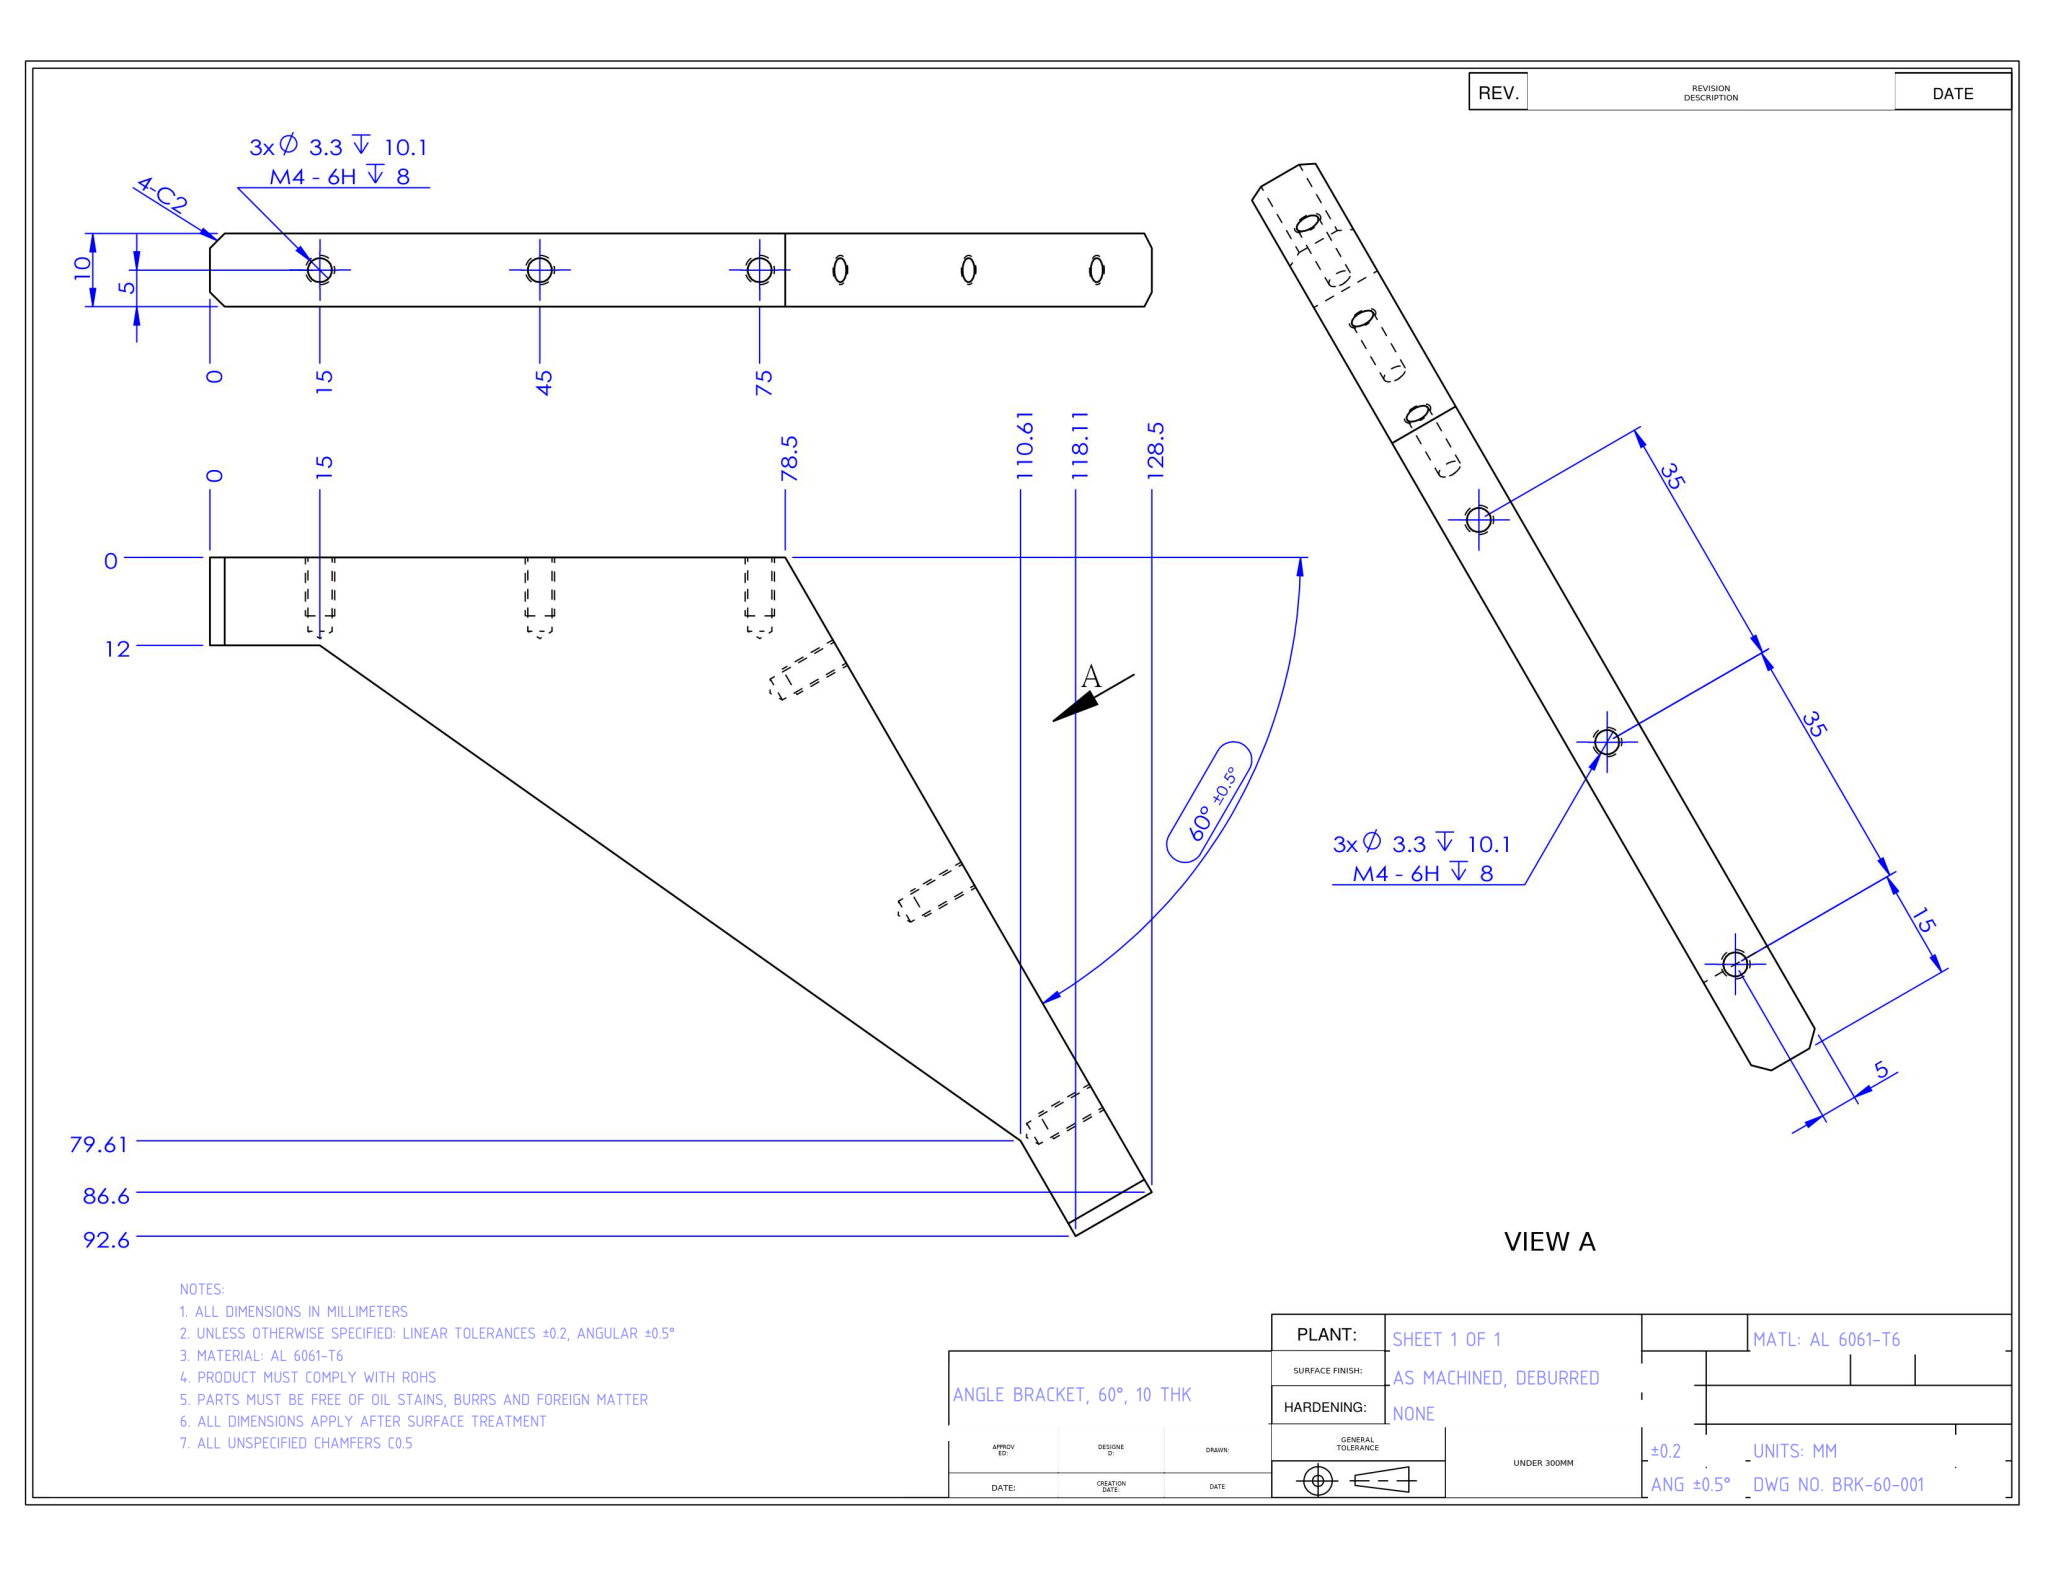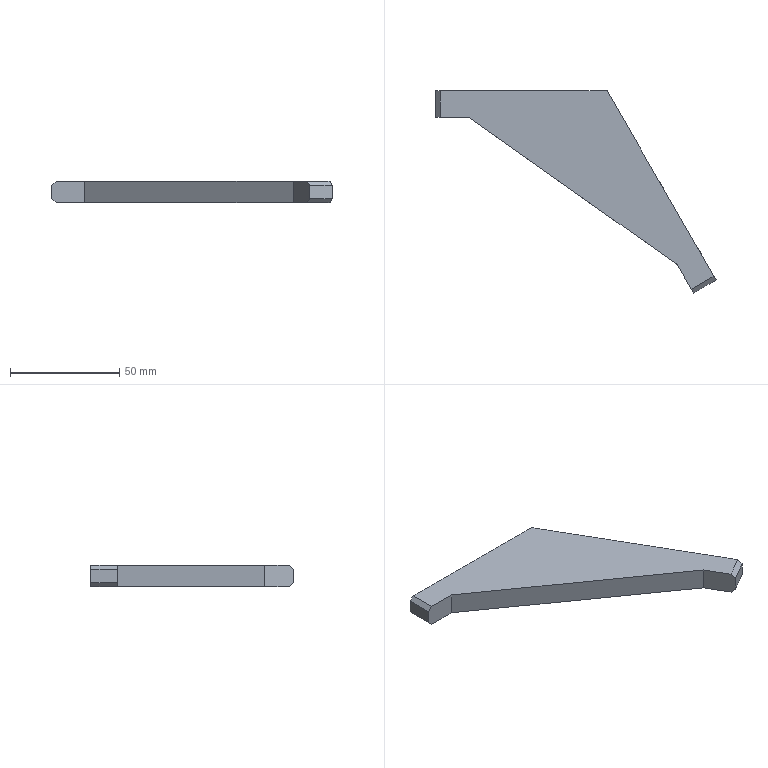Part | NX | mm | 1 solid | 37 faces | box 128.5 x 92.6 x 10 mm | volume 39082 mm3 | plane 13 | cylinder 12 | cone 12 | commonest cylinder face diameters 3.3 x12